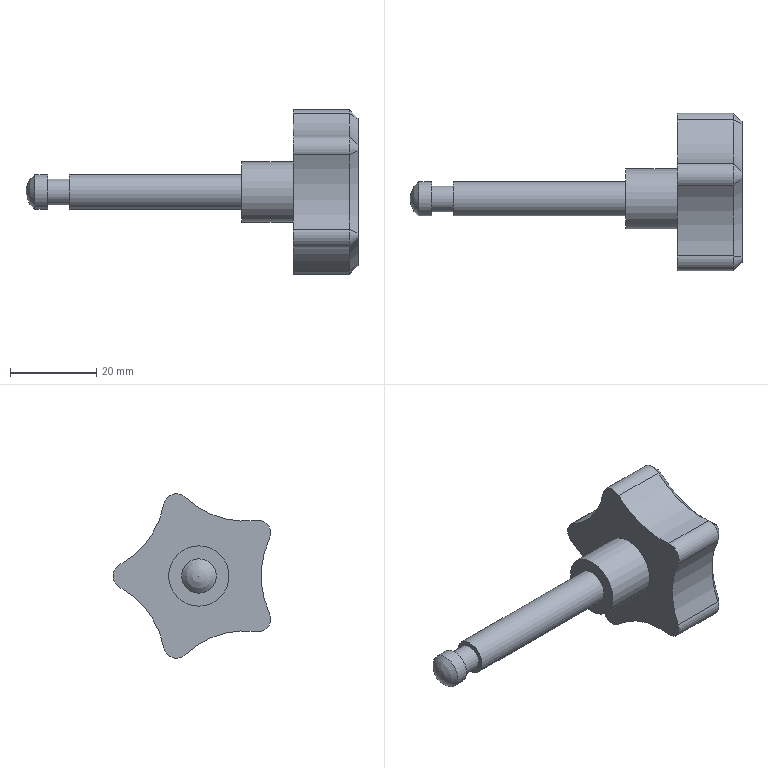Component | NX | HEX_HANDLE | 1 solid | 30 faces | volume 16927 mm3 | cylinder 14 | cone 10 | plane 5 | sphere 1 | commonest cylinder face diameters 6 x6 40 x5 8 x2 14 x1